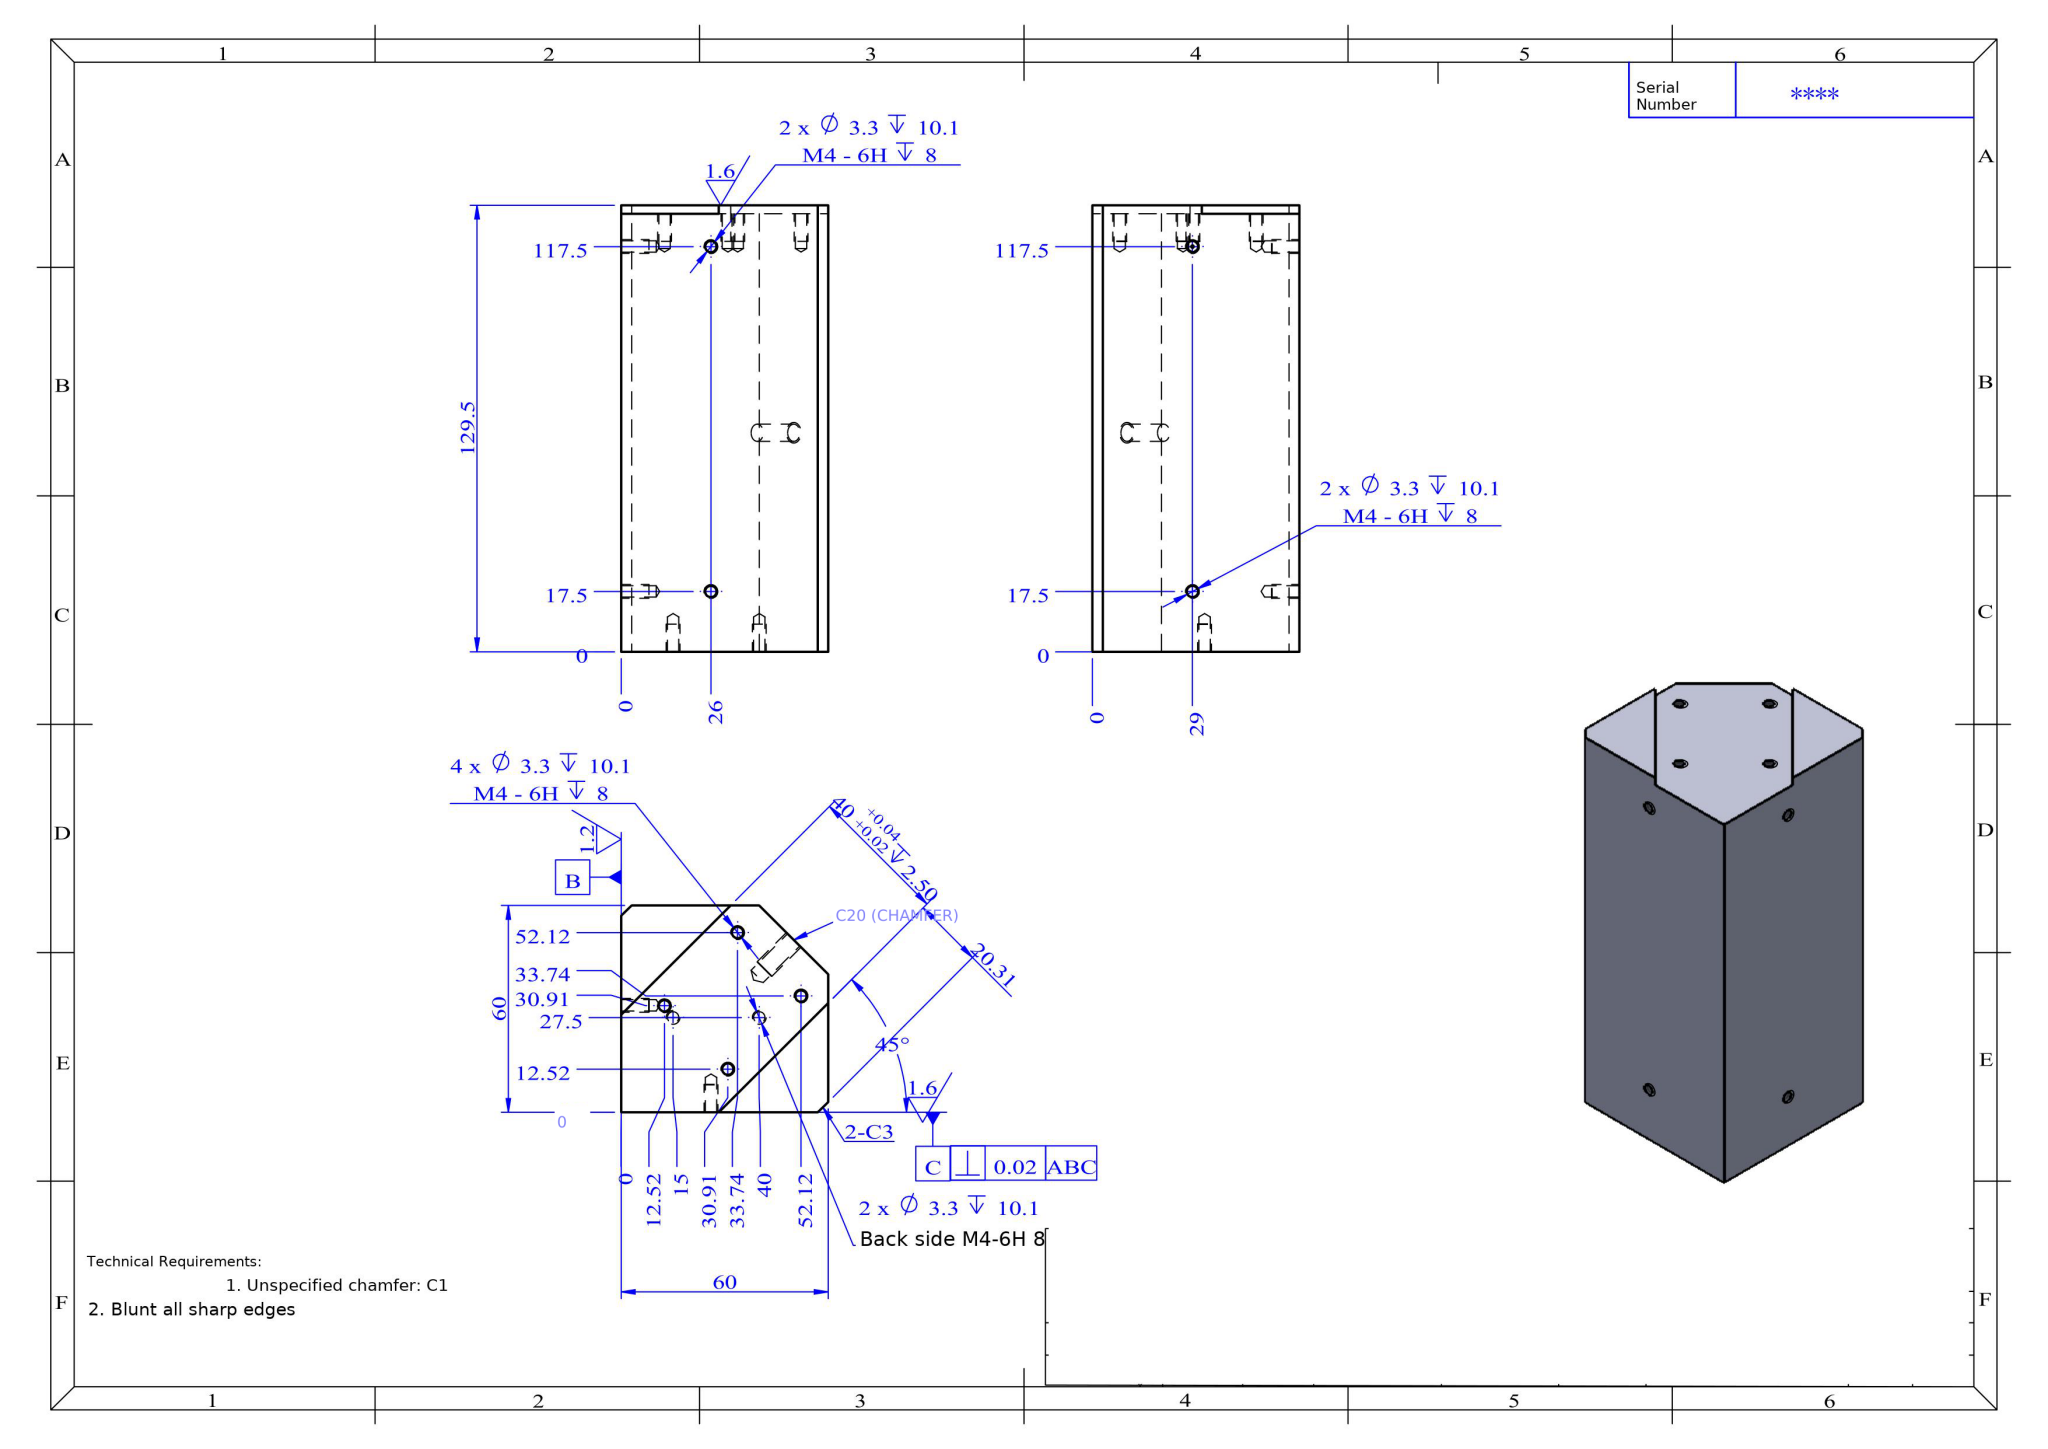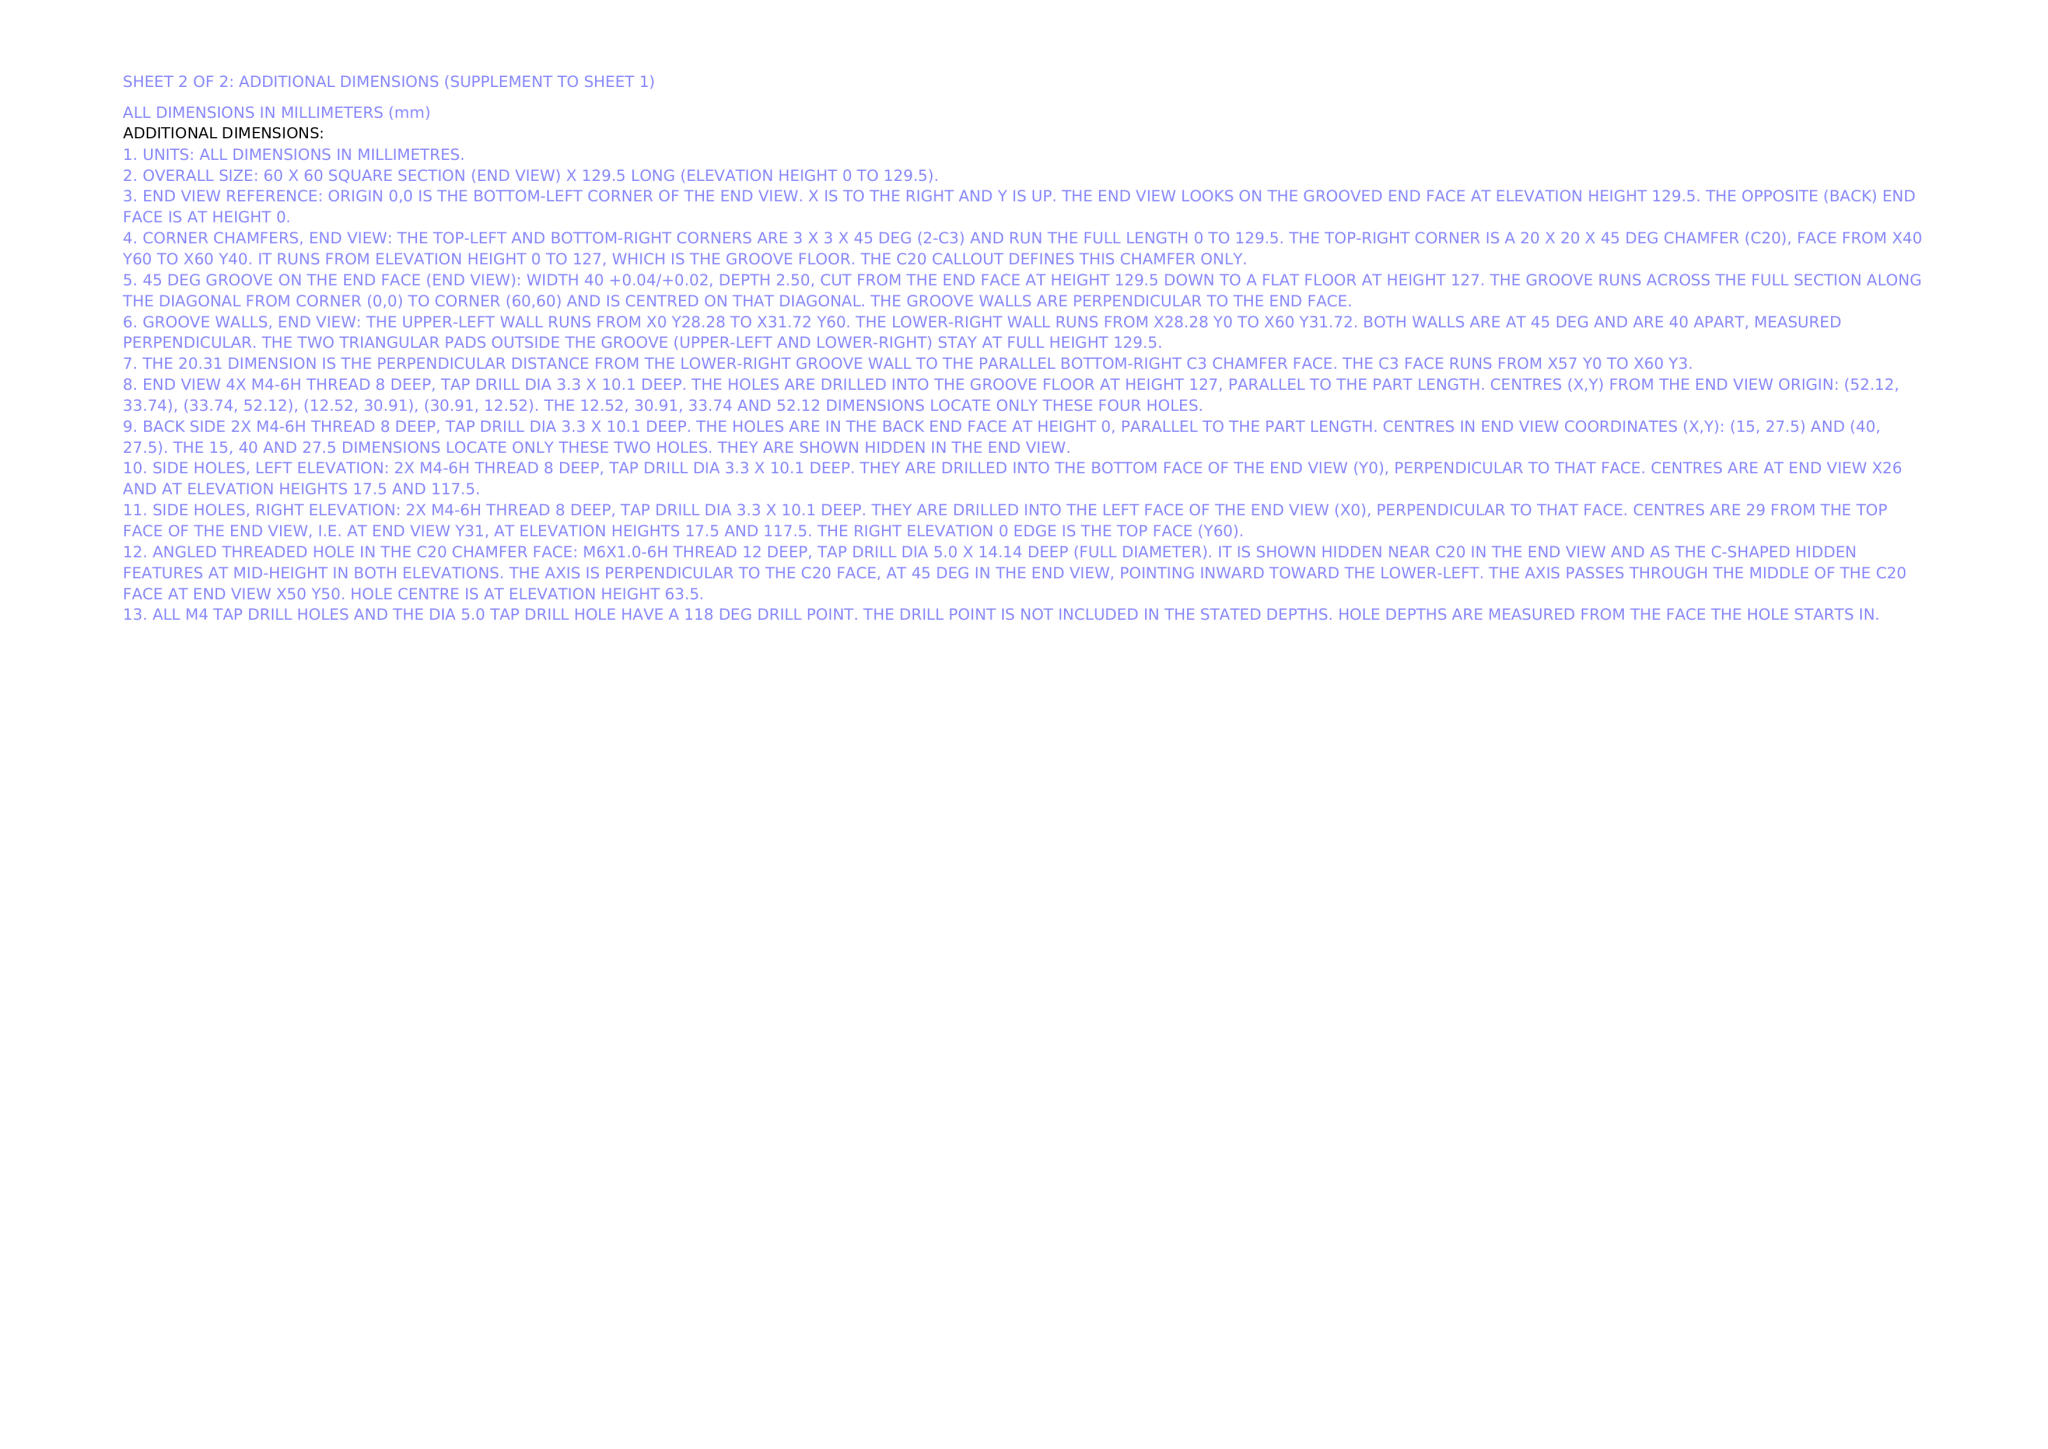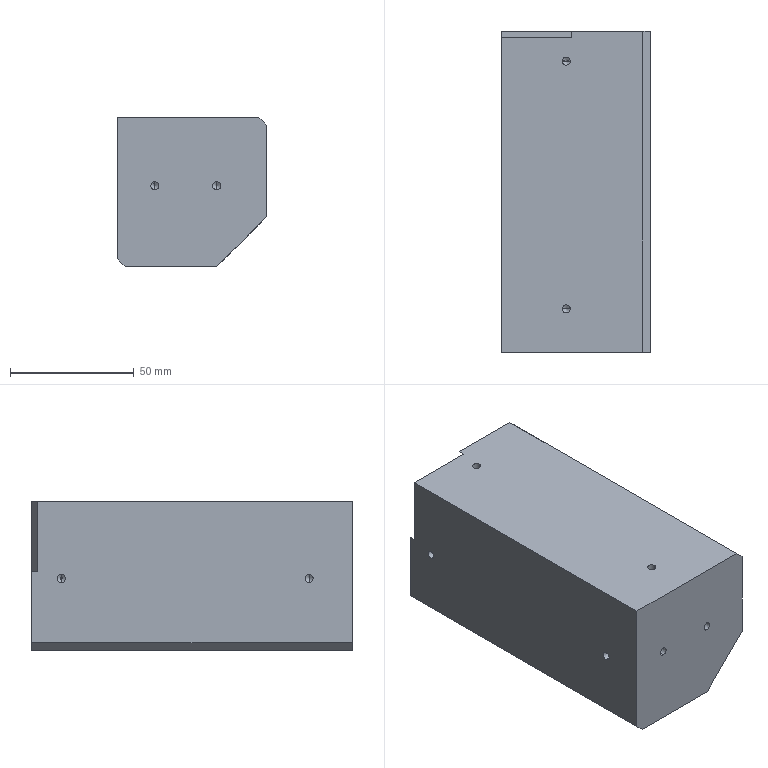Part | NX | mm | 1 solid | 57 faces | box 60 x 129.5 x 60 mm | volume 431953 mm3 | cylinder 22 | cone 22 | plane 13 | commonest cylinder face diameters 3.3 x20 5 x2